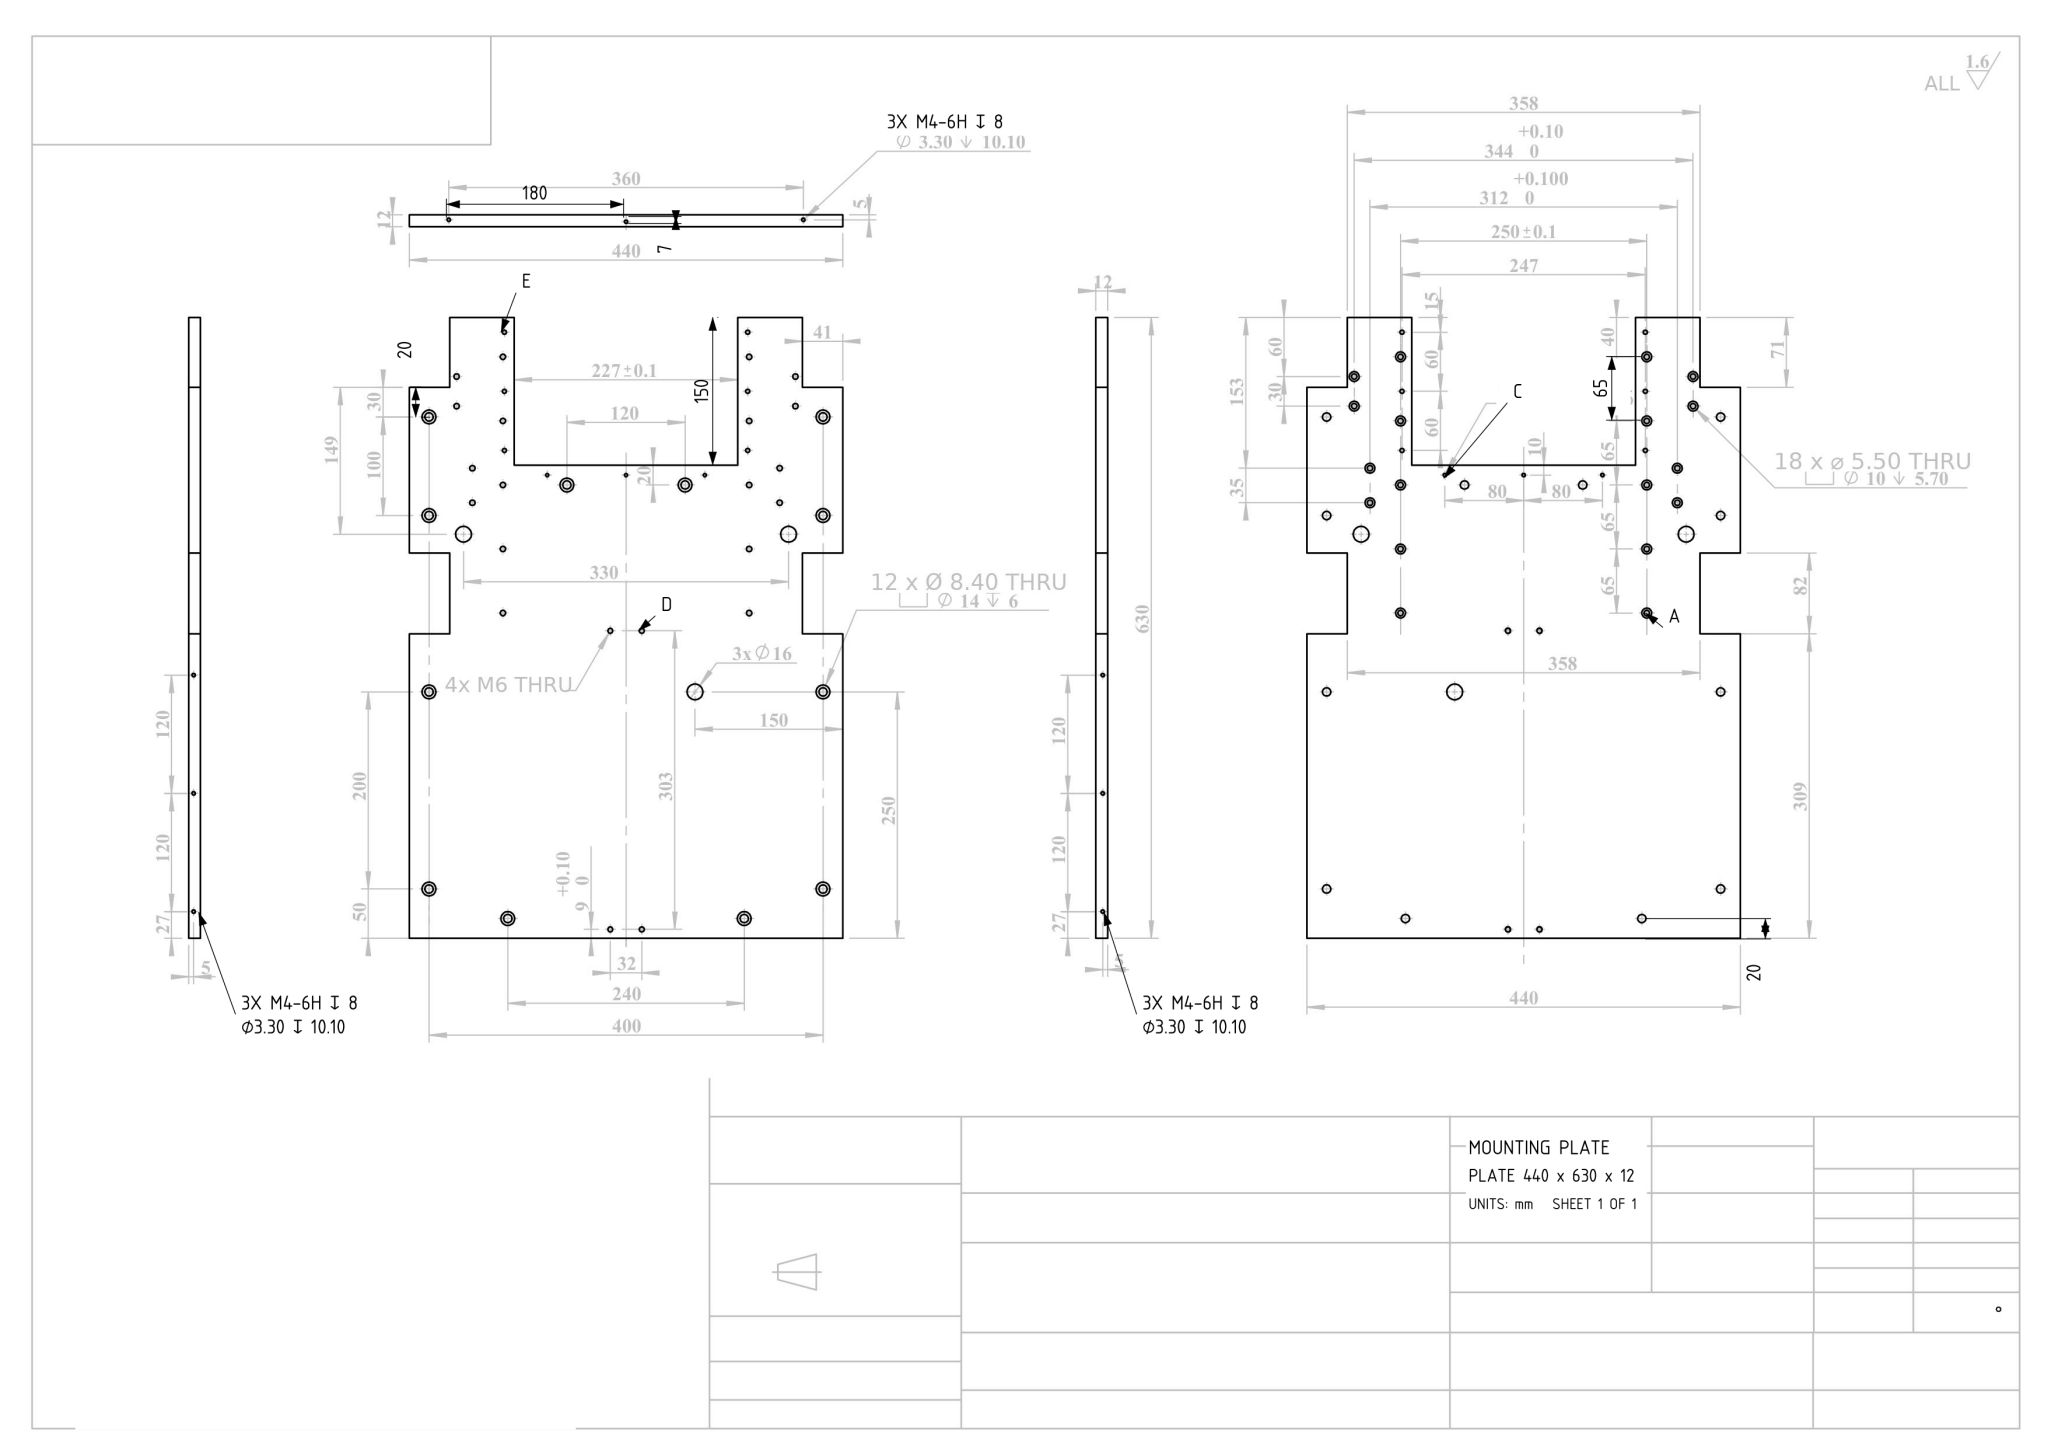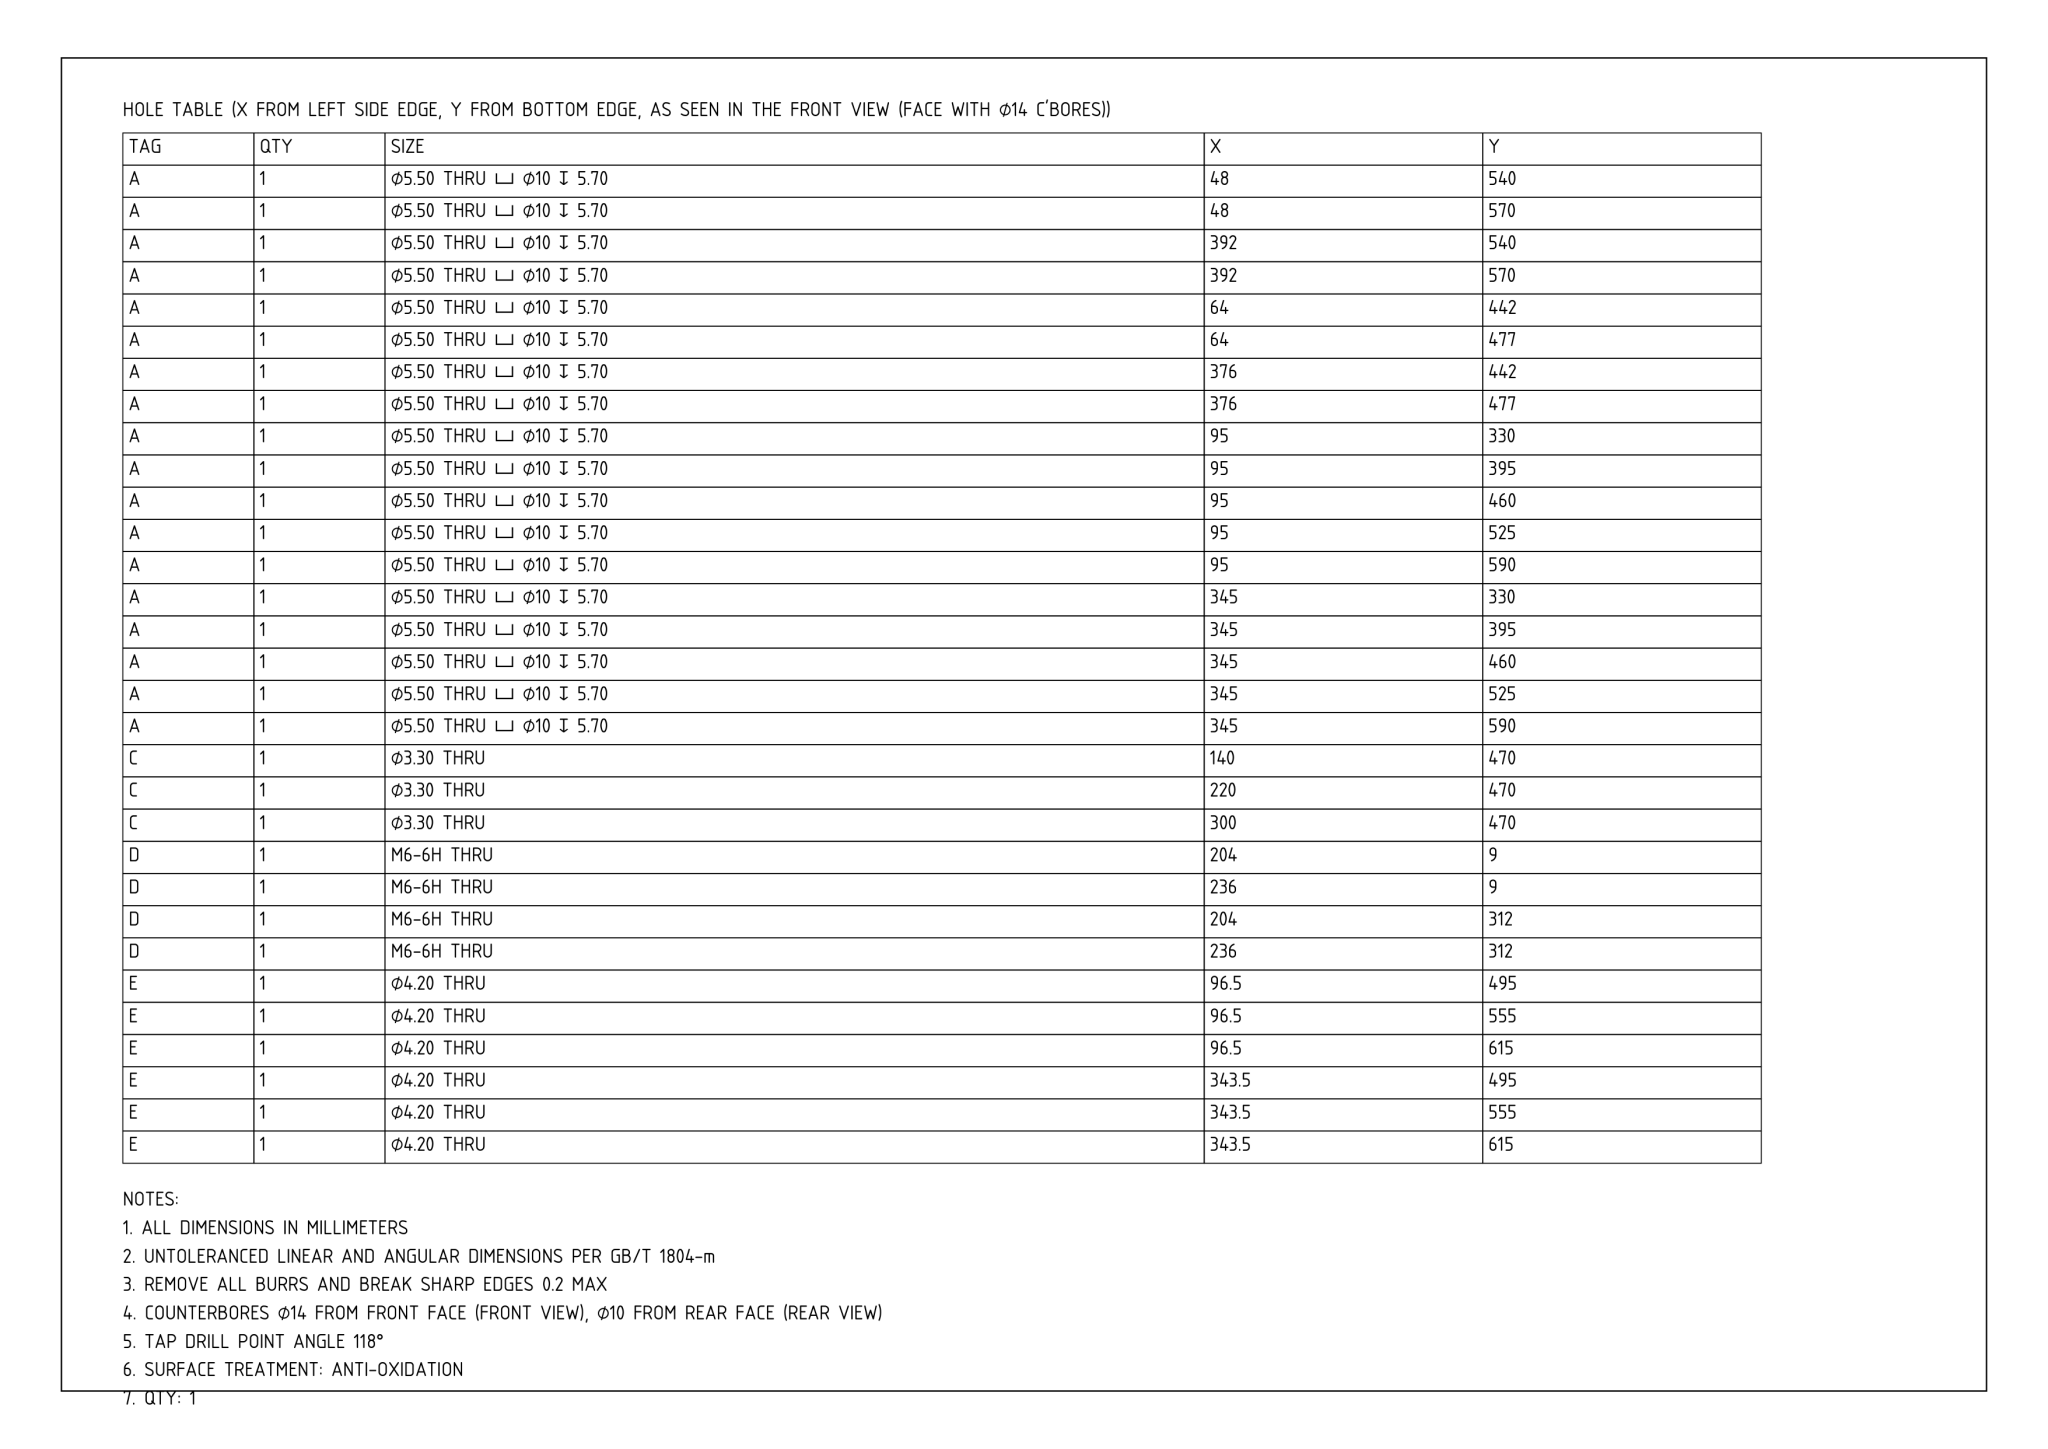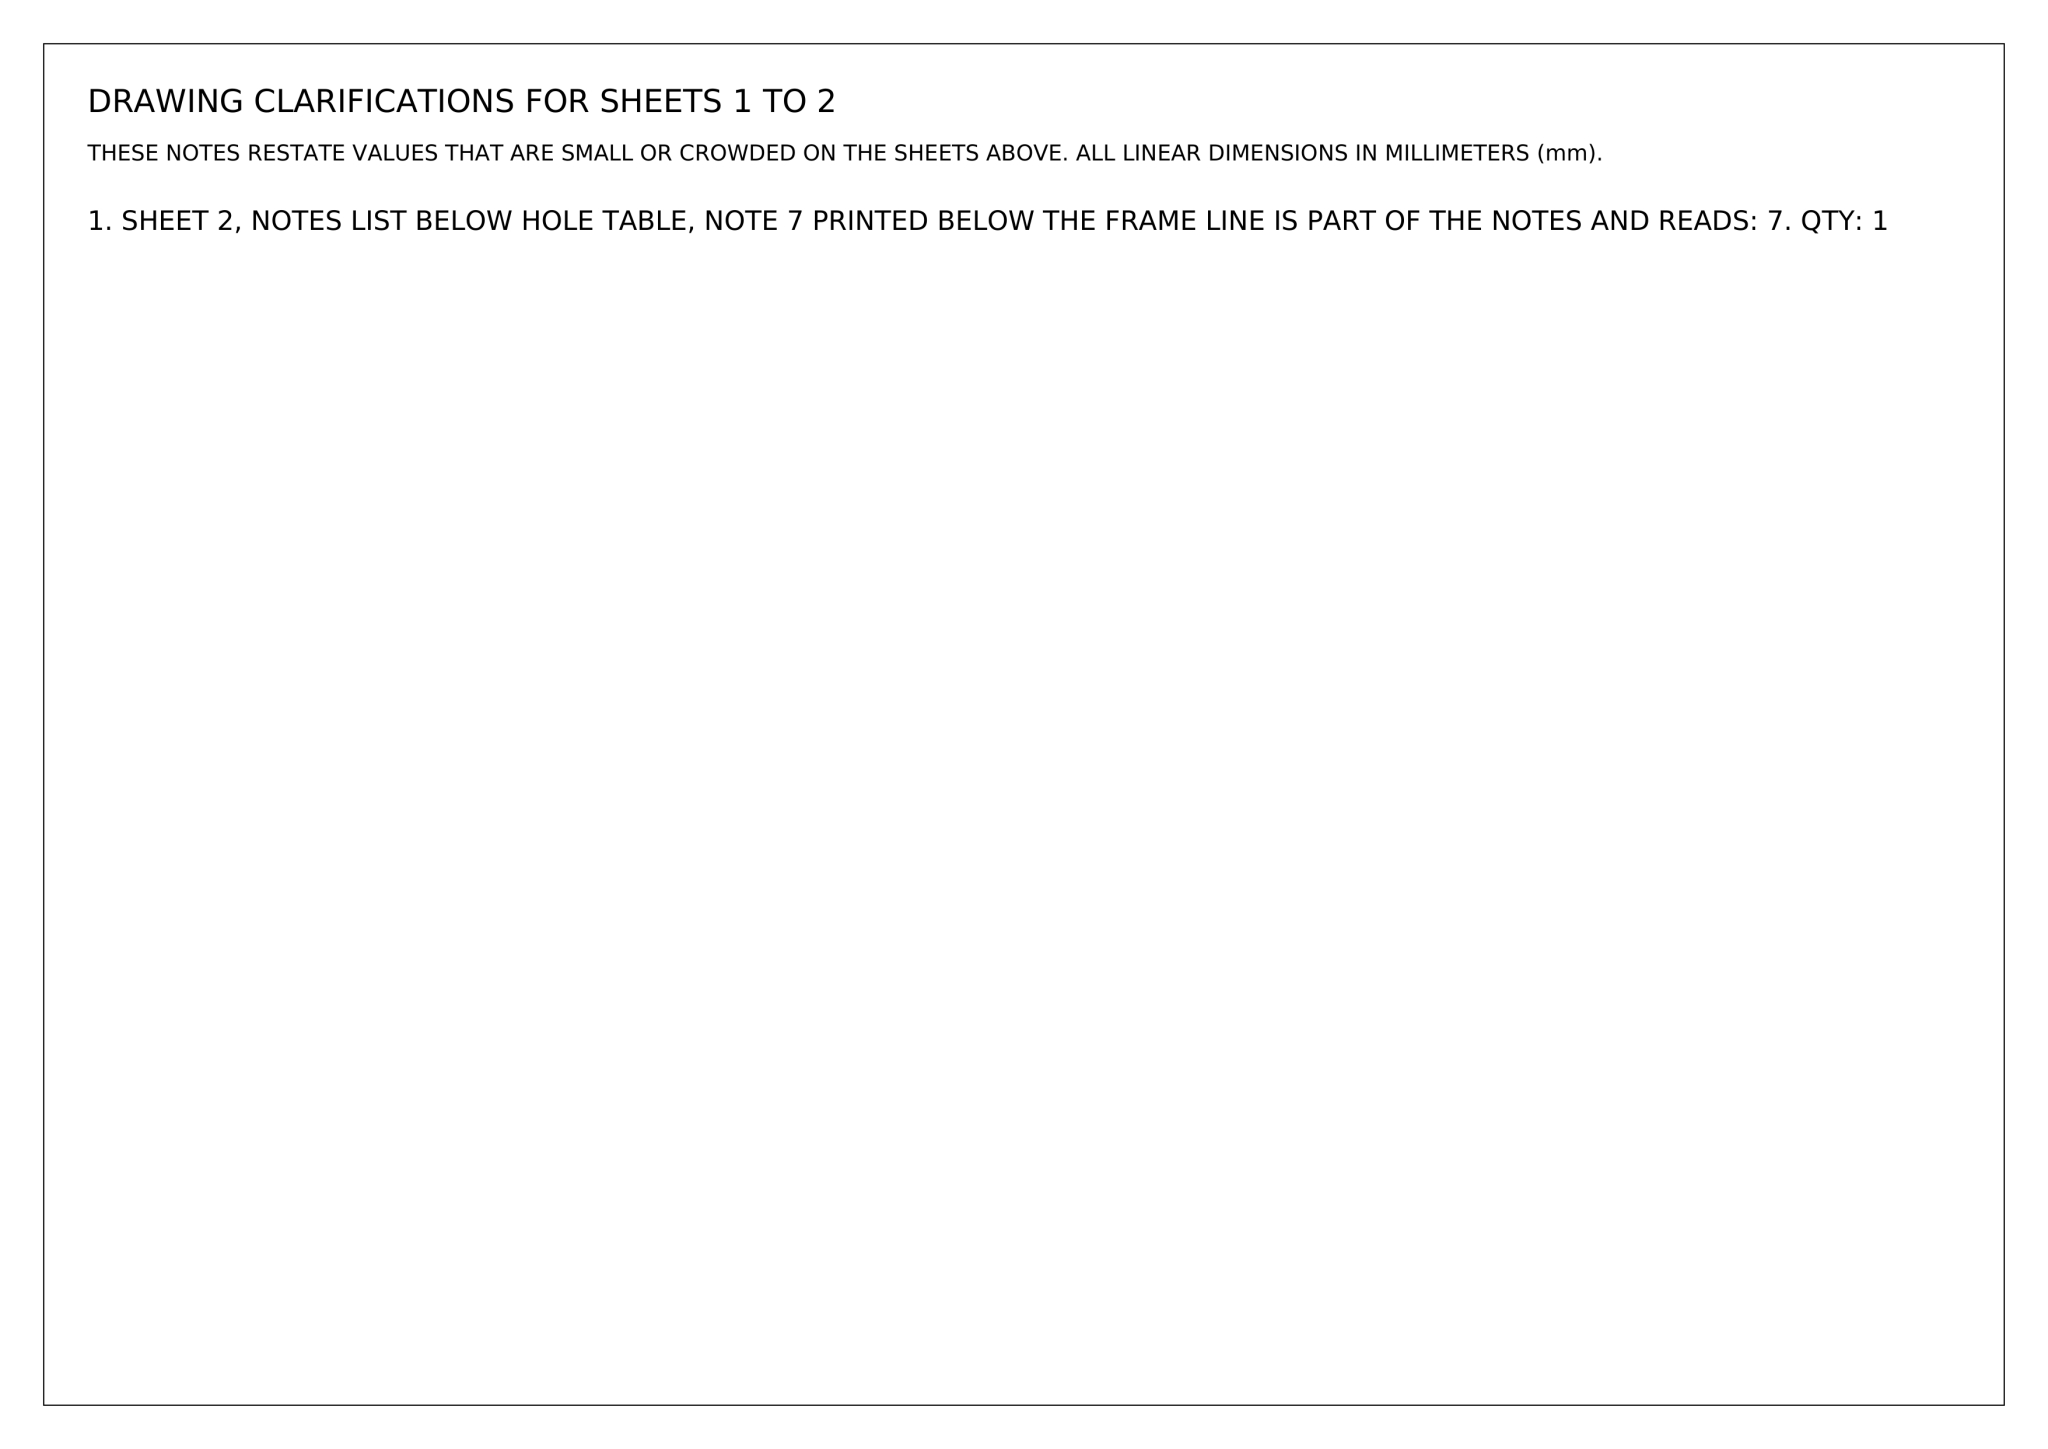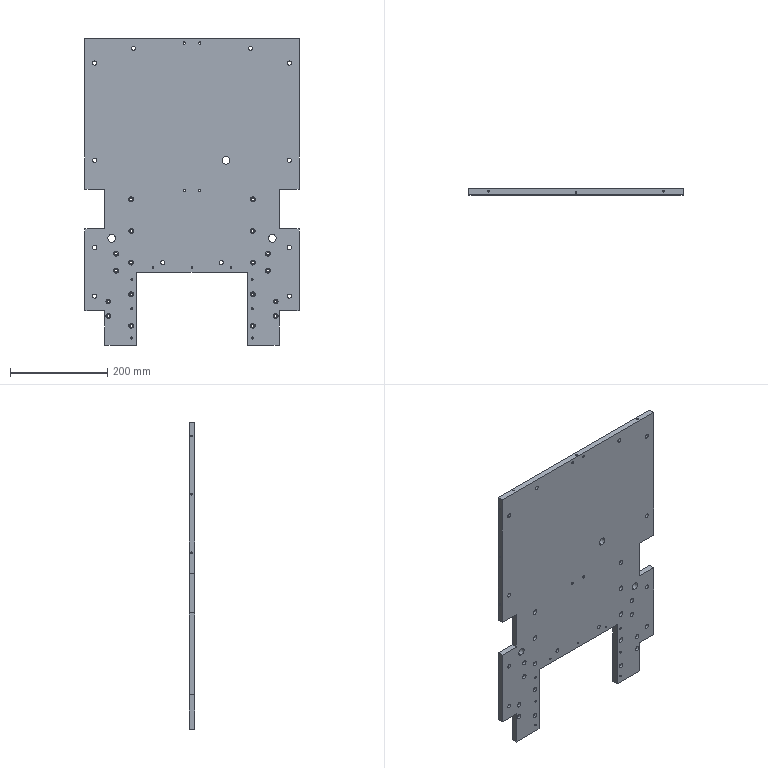Part | NX | mm | 1 solid | 242 faces | box 440 x 12 x 630 mm | volume 2731133 mm3 | cylinder 170 | plane 54 | cone 18 | commonest cylinder face diameters 10 x36 5.5 x36 14 x24 8.4 x24 3.3 x24 4.2 x12 5 x8 16 x6